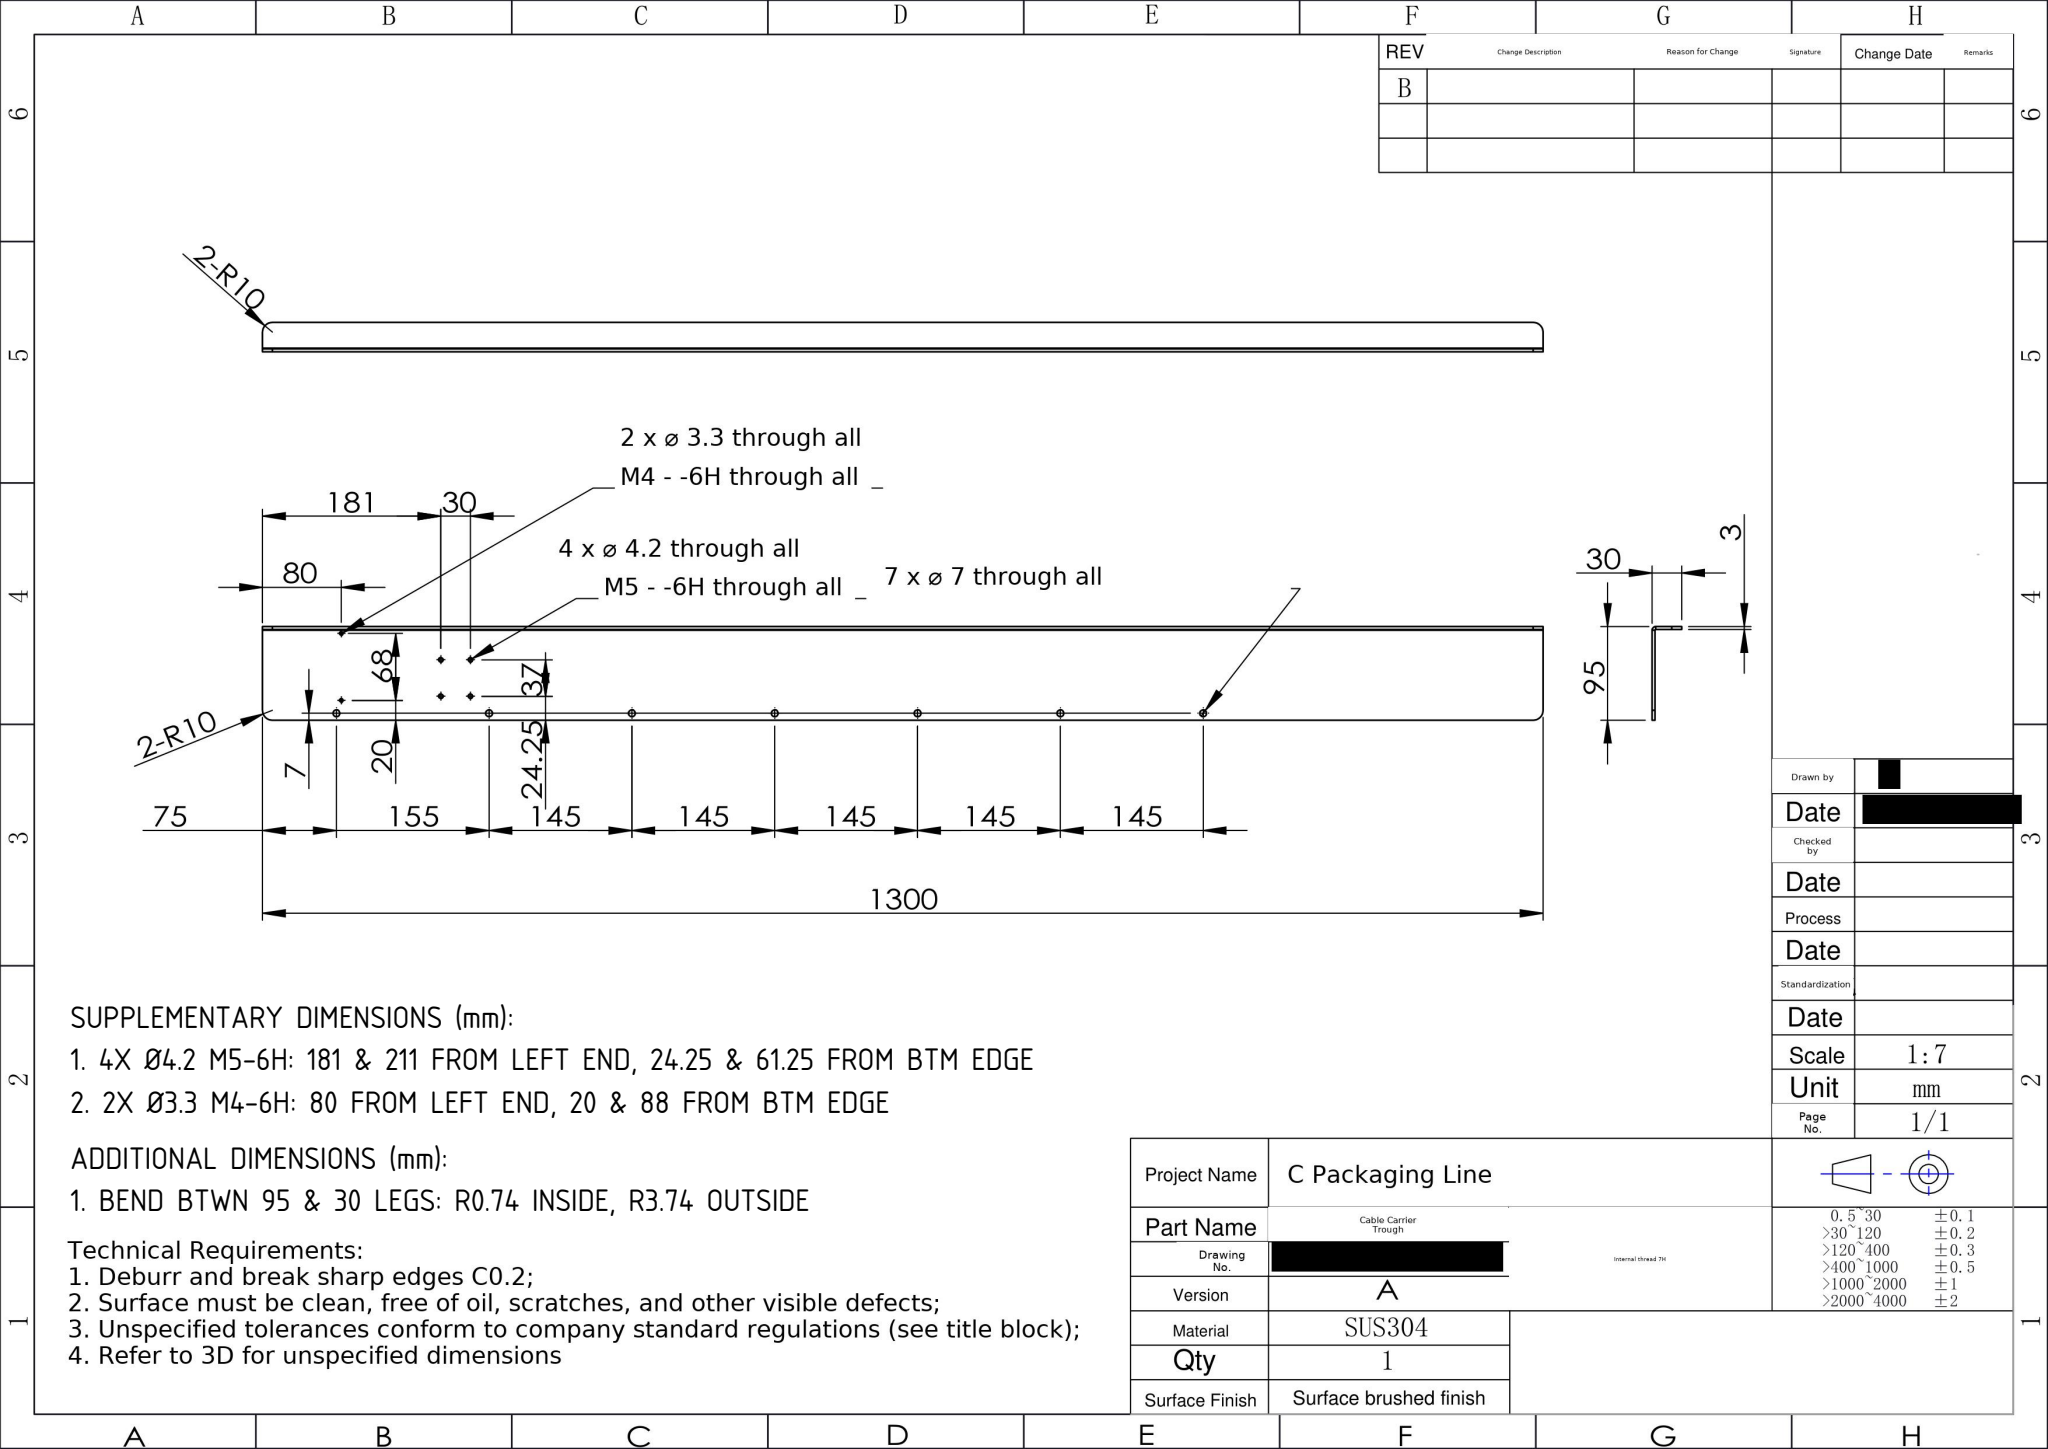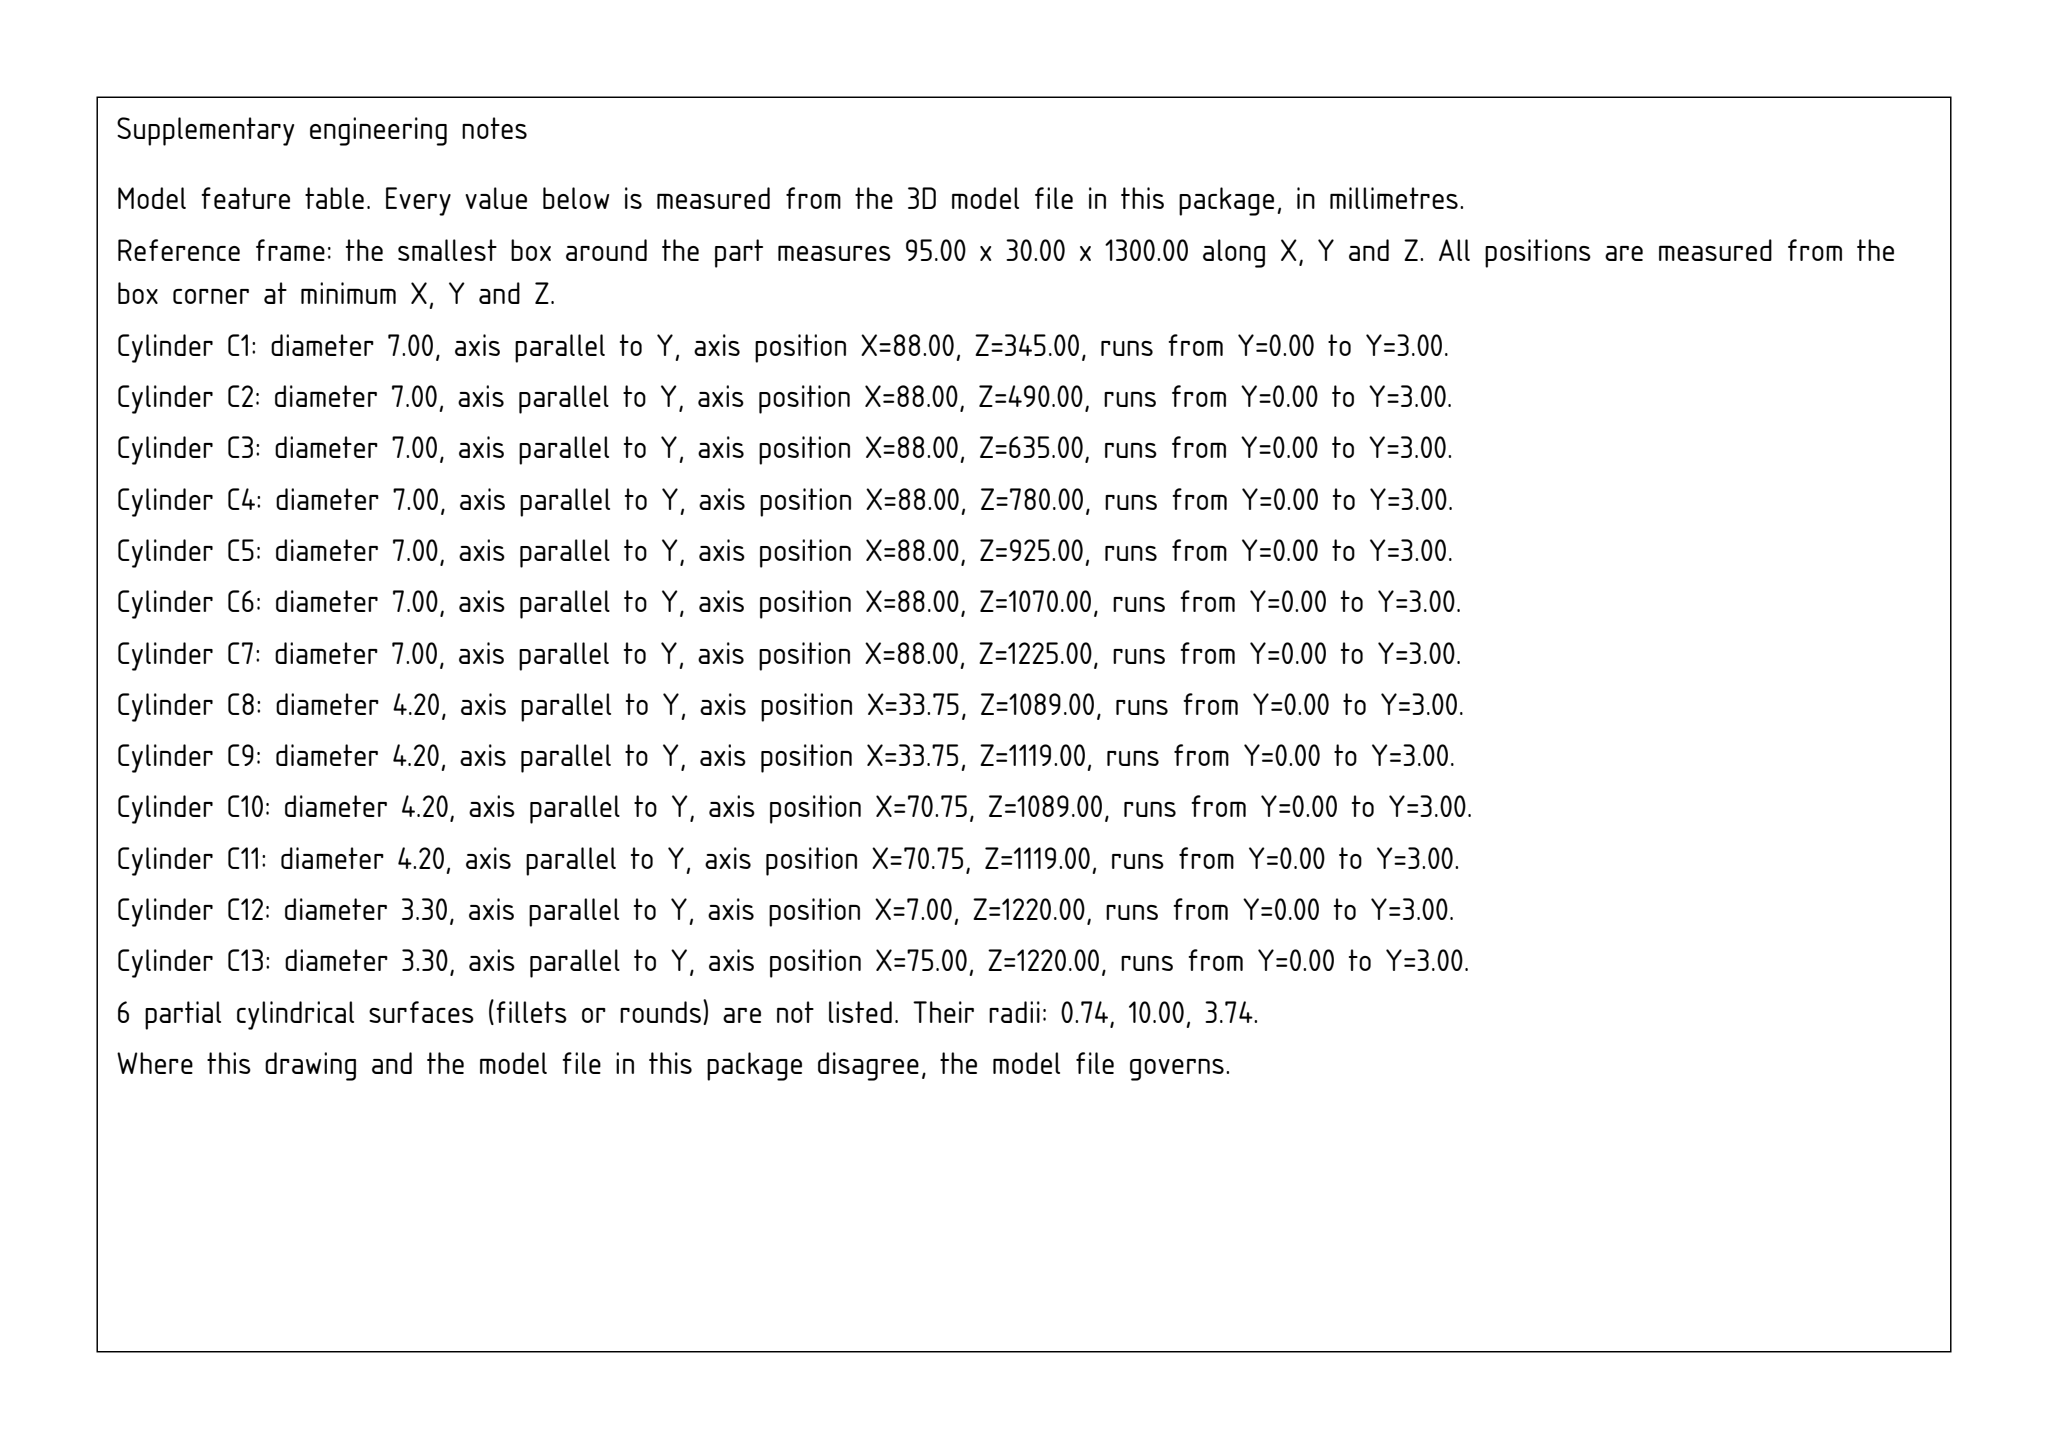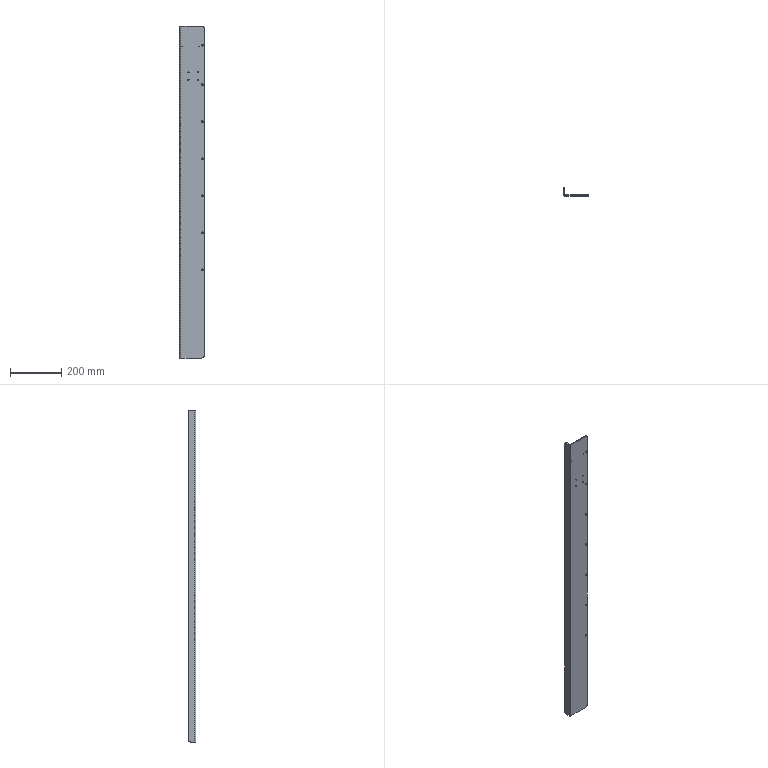Part | SolidWorks | mm | 1 solid | 44 faces | box 95 x 30 x 1300 mm | volume 470773 mm3 | cylinder 32 | plane 12 | commonest cylinder face diameters 7 x14 4.2 x8 3.3 x4 20 x4 1.473 x1 7.473 x1